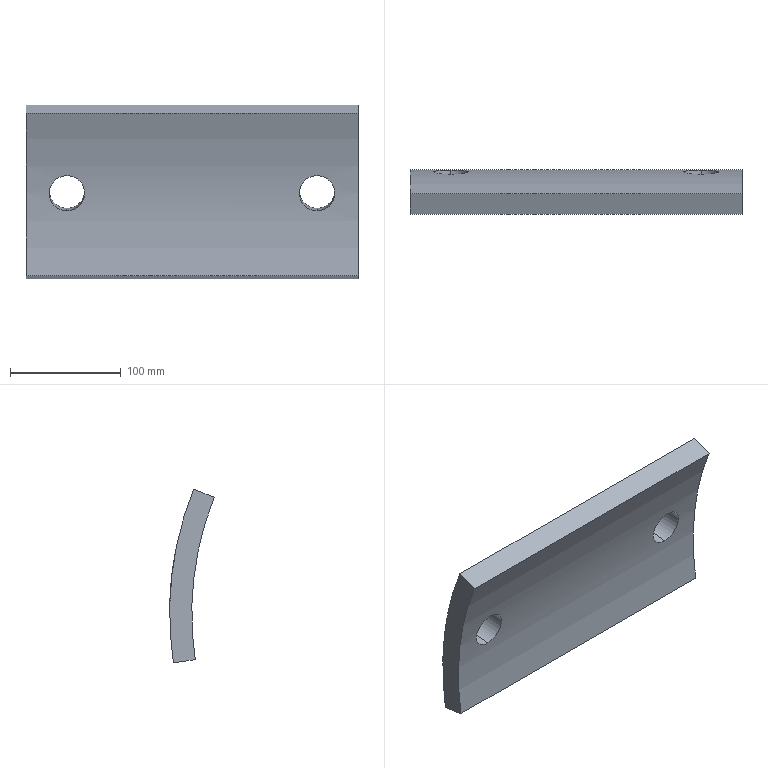Component | SolidWorks | Donja ploca spone-2 | 1 solid | 10 faces | box 300 x 40.3 x 157.04 mm | volume 895871 mm3 | cylinder 6 | plane 4 | commonest cylinder face diameters 32 x4 601 x1 561 x1
build123d program:
from build123d import *

# Parameters (mm, degrees)
BOSS_EXTRUDE1_DEPTH      = 150
BOSS_EXTRUDE1_DEPTH_BACK = 150
CUT_EXTRUDE3_DEPTH       = 171.734
CUT_EXTRUDE3_DEPTH_BACK  = 171.734
SKETCH2_R                = 16


with BuildPart() as part:
    # Sketch1 → Boss-Extrude1 (new, two sides: drawn at the far end of the back side and taken through both)
    with BuildSketch(Plane(origin=(0, 0, 0), x_dir=(0, 0, -1), z_dir=(1, 0, 0)).offset(-BOSS_EXTRUDE1_DEPTH_BACK)):
        with BuildLine():
            Line((-73.797, -9.882), (-79.058, 9.414))
            ThreePointArc((-79.058, 9.414), (0, 20), (79.058, 9.414))
            Line((79.058, 9.414), (73.797, -9.882))
            ThreePointArc((73.797, -9.882), (0, 0), (-73.797, -9.882))
        make_face()
    extrude(amount=BOSS_EXTRUDE1_DEPTH + BOSS_EXTRUDE1_DEPTH_BACK)

    # Sketch2 → Cut-Extrude3 (cut, two sides: drawn at the far end of the back side and taken through both)
    with BuildSketch(Plane(origin=(0, 0, 0), x_dir=(1, 0, 0), z_dir=(0, 1, 0)).offset(-CUT_EXTRUDE3_DEPTH_BACK)):
        with Locations(Location((113, 0, 0), (0, 0, 90))):
            Circle(SKETCH2_R)
        with Locations(Location((-113, 0, 0), (0, 0, 90))):
            Circle(SKETCH2_R)
    extrude(amount=CUT_EXTRUDE3_DEPTH + CUT_EXTRUDE3_DEPTH_BACK, mode=Mode.SUBTRACT)


solid = part.part

# Placed as in the assembly
solid = solid.moved(Location((-80, 278.597, 32.617), (6.678, 0, 0)))
STEP:
#1=CARTESIAN_POINT('',(-7.598,11.661,1.999));
#2=VERTEX_POINT('',#1);
#3=CARTESIAN_POINT('',(-7.598,11.807,0.7481));
#4=VERTEX_POINT('',#3);
#5=CARTESIAN_POINT('',(-7.598,11.661,1.999));
#6=CARTESIAN_POINT('',(-7.64,11.661,1.999));
#7=CARTESIAN_POINT('',(-7.68,11.661,1.995));
#8=CARTESIAN_POINT('',(-7.741,11.663,1.984));
#9=CARTESIAN_POINT('',(-7.762,11.664,1.979));
#10=CARTESIAN_POINT('',(-7.801,11.666,1.967));
#11=CARTESIAN_POINT('',(-7.84,11.668,1.953));
#12=CARTESIAN_POINT('',(-7.877,11.671,1.936));
#13=CARTESIAN_POINT('',(-7.913,11.674,1.917));
#14=CARTESIAN_POINT('',(-7.931,11.676,1.906));
#15=CARTESIAN_POINT('',(-7.983,11.682,1.872));
#16=CARTESIAN_POINT('',(-8.014,11.686,1.846));
#17=CARTESIAN_POINT('',(-8.058,11.693,1.803));
#18=CARTESIAN_POINT('',(-8.072,11.695,1.788));
#19=CARTESIAN_POINT('',(-8.098,11.7,1.756));
#20=CARTESIAN_POINT('',(-8.111,11.702,1.74));
#21=CARTESIAN_POINT('',(-8.145,11.71,1.689));
#22=CARTESIAN_POINT('',(-8.164,11.715,1.653));
#23=CARTESIAN_POINT('',(-8.188,11.723,1.597));
#24=CARTESIAN_POINT('',(-8.195,11.725,1.577));
#25=CARTESIAN_POINT('',(-8.207,11.73,1.538));
#26=CARTESIAN_POINT('',(-8.212,11.733,1.518));
#27=CARTESIAN_POINT('',(-8.224,11.741,1.458));
#28=CARTESIAN_POINT('',(-8.228,11.746,1.417));
#29=CARTESIAN_POINT('',(-8.228,11.753,1.356));
#30=CARTESIAN_POINT('',(-8.227,11.755,1.335));
#31=CARTESIAN_POINT('',(-8.223,11.76,1.294));
#32=CARTESIAN_POINT('',(-8.22,11.762,1.274));
#33=CARTESIAN_POINT('',(-8.212,11.766,1.234));
#34=CARTESIAN_POINT('',(-8.207,11.768,1.214));
#35=CARTESIAN_POINT('',(-8.195,11.772,1.175));
#36=CARTESIAN_POINT('',(-8.188,11.774,1.155));
#37=CARTESIAN_POINT('',(-8.165,11.78,1.098));
#38=CARTESIAN_POINT('',(-8.145,11.783,1.062));
#39=CARTESIAN_POINT('',(-8.111,11.787,1.011));
#40=CARTESIAN_POINT('',(-8.099,11.789,0.9945));
#41=CARTESIAN_POINT('',(-8.073,11.792,0.9624));
#42=CARTESIAN_POINT('',(-8.059,11.793,0.9472));
#43=CARTESIAN_POINT('',(-8.015,11.796,0.9036));
#44=CARTESIAN_POINT('',(-7.983,11.798,0.8776));
#45=CARTESIAN_POINT('',(-7.932,11.801,0.8431));
#46=CARTESIAN_POINT('',(-7.914,11.801,0.8324));
#47=CARTESIAN_POINT('',(-7.878,11.803,0.8129));
#48=CARTESIAN_POINT('',(-7.84,11.804,0.7954));
#49=CARTESIAN_POINT('',(-7.802,11.805,0.7815));
#50=CARTESIAN_POINT('',(-7.762,11.806,0.7695));
#51=CARTESIAN_POINT('',(-7.742,11.806,0.7644));
#52=CARTESIAN_POINT('',(-7.681,11.807,0.7522));
#53=CARTESIAN_POINT('',(-7.64,11.807,0.7481));
#54=CARTESIAN_POINT('',(-7.598,11.807,0.7481));
#55=B_SPLINE_CURVE_WITH_KNOTS('',3,(#5,#6,#7,#8,#9,#10,#11,#12,#13,#14,#15,#16,#17,#18,#19,#20,#21,#22,#23,#24,#25,#26,#27,#28,#29,#30,#31,#32,#33,#34,#35,#36,#37,#38,#39,#40,#41,#42,#43,#44,#45,#46,#47,#48,#49,#50,#51,#52,#53,#54),.UNSPECIFIED.,.F.,.F.,(4,2,2,1,2,2,2,2,2,2,2,2,2,2,2,2,2,2,2,2,2,2,1,2,2,4),(0.05003,0.05316,0.05472,0.05628,0.05785,0.05941,0.06254,0.0641,0.06566,0.06879,0.07035,0.07192,0.07504,0.07661,0.07817,0.07973,0.0813,0.08442,0.08598,0.08755,0.09067,0.09224,0.0938,0.09536,0.09693,0.1001),.UNSPECIFIED.);
#56=EDGE_CURVE('',#2,#4,#55,.T.);
#57=ORIENTED_EDGE('',*,*,#56,.F.);
#58=CARTESIAN_POINT('',(-7.598,10.877,1.908));
#59=VERTEX_POINT('',#58);
#60=CARTESIAN_POINT('',(-7.598,11.677,2.001));
#61=DIRECTION('',(0.,-0.9932,-0.1163));
#62=VECTOR('',#61,39.37);
#63=LINE('',#60,#62);
#64=EDGE_CURVE('',#2,#59,#63,.T.);
#65=ORIENTED_EDGE('',*,*,#64,.T.);
#66=CARTESIAN_POINT('',(-7.598,11.024,0.6564));
#67=VERTEX_POINT('',#66);
#68=CARTESIAN_POINT('',(-7.598,11.024,0.6564));
#69=CARTESIAN_POINT('',(-7.64,11.024,0.6564));
#70=CARTESIAN_POINT('',(-7.681,11.024,0.6605));
#71=CARTESIAN_POINT('',(-7.741,11.023,0.6725));
#72=CARTESIAN_POINT('',(-7.761,11.023,0.6775));
#73=CARTESIAN_POINT('',(-7.801,11.022,0.6895));
#74=CARTESIAN_POINT('',(-7.821,11.021,0.6965));
#75=CARTESIAN_POINT('',(-7.878,11.02,0.7202));
#76=CARTESIAN_POINT('',(-7.914,11.019,0.7396));
#77=CARTESIAN_POINT('',(-7.965,11.016,0.7738));
#78=CARTESIAN_POINT('',(-7.982,11.015,0.7862));
#79=CARTESIAN_POINT('',(-8.014,11.013,0.8125));
#80=CARTESIAN_POINT('',(-8.029,11.012,0.8263));
#81=CARTESIAN_POINT('',(-8.073,11.009,0.8698));
#82=CARTESIAN_POINT('',(-8.099,11.007,0.9014));
#83=CARTESIAN_POINT('',(-8.134,11.002,0.9529));
#84=CARTESIAN_POINT('',(-8.144,11.001,0.9707));
#85=CARTESIAN_POINT('',(-8.164,10.997,1.007));
#86=CARTESIAN_POINT('',(-8.181,10.994,1.044));
#87=CARTESIAN_POINT('',(-8.195,10.99,1.082));
#88=CARTESIAN_POINT('',(-8.207,10.986,1.122));
#89=CARTESIAN_POINT('',(-8.212,10.984,1.142));
#90=CARTESIAN_POINT('',(-8.224,10.978,1.202));
#91=CARTESIAN_POINT('',(-8.228,10.973,1.243));
#92=CARTESIAN_POINT('',(-8.228,10.966,1.304));
#93=CARTESIAN_POINT('',(-8.227,10.964,1.325));
#94=CARTESIAN_POINT('',(-8.223,10.959,1.366));
#95=CARTESIAN_POINT('',(-8.22,10.956,1.386));
#96=CARTESIAN_POINT('',(-8.208,10.948,1.446));
#97=CARTESIAN_POINT('',(-8.196,10.943,1.485));
#98=CARTESIAN_POINT('',(-8.173,10.935,1.542));
#99=CARTESIAN_POINT('',(-8.164,10.932,1.561));
#100=CARTESIAN_POINT('',(-8.144,10.927,1.597));
#101=CARTESIAN_POINT('',(-8.134,10.925,1.614));
#102=CARTESIAN_POINT('',(-8.099,10.917,1.665));
#103=CARTESIAN_POINT('',(-8.073,10.912,1.696));
#104=CARTESIAN_POINT('',(-8.015,10.903,1.754));
#105=CARTESIAN_POINT('',(-7.983,10.899,1.78));
#106=CARTESIAN_POINT('',(-7.932,10.893,1.814));
#107=CARTESIAN_POINT('',(-7.914,10.892,1.825));
#108=CARTESIAN_POINT('',(-7.877,10.888,1.844));
#109=CARTESIAN_POINT('',(-7.859,10.887,1.853));
#110=CARTESIAN_POINT('',(-7.801,10.883,1.876));
#111=CARTESIAN_POINT('',(-7.762,10.881,1.888));
#112=CARTESIAN_POINT('',(-7.701,10.879,1.9));
#113=CARTESIAN_POINT('',(-7.681,10.878,1.903));
#114=CARTESIAN_POINT('',(-7.64,10.877,1.907));
#115=CARTESIAN_POINT('',(-7.619,10.877,1.908));
#116=CARTESIAN_POINT('',(-7.598,10.877,1.908));
#117=B_SPLINE_CURVE_WITH_KNOTS('',3,(#68,#69,#70,#71,#72,#73,#74,#75,#76,#77,#78,#79,#80,#81,#82,#83,#84,#85,#86,#87,#88,#89,#90,#91,#92,#93,#94,#95,#96,#97,#98,#99,#100,#101,#102,#103,#104,#105,#106,#107,#108,#109,#110,#111,#112,#113,#114,#115,#116),.UNSPECIFIED.,.F.,.F.,(4,2,2,2,2,2,2,2,2,1,2,2,2,2,2,2,2,2,2,2,2,2,2,2,4),(0.,0.003127,0.004691,0.006254,0.009381,0.01094,0.01251,0.01564,0.0172,0.01876,0.02033,0.02189,0.02502,0.02658,0.02814,0.03127,0.03283,0.0344,0.03753,0.04065,0.04222,0.04378,0.04691,0.04847,0.05003),.UNSPECIFIED.);
#118=EDGE_CURVE('',#67,#59,#117,.T.);
#119=ORIENTED_EDGE('',*,*,#118,.F.);
#120=CARTESIAN_POINT('',(-7.598,11.824,0.7501));
#121=DIRECTION('',(0.,-0.9932,-0.1163));
#122=VECTOR('',#121,39.37);
#123=LINE('',#120,#122);
#124=EDGE_CURVE('',#4,#67,#123,.T.);
#125=ORIENTED_EDGE('',*,*,#124,.F.);
#126=EDGE_LOOP('',(#57,#65,#119,#125));
#127=FACE_OUTER_BOUND('',#126,.T.);
#128=CARTESIAN_POINT('',(-7.598,11.75,1.376));
#129=DIRECTION('',(0.,-0.9932,-0.1163));
#130=DIRECTION('',(0.,0.1163,-0.9932));
#131=AXIS2_PLACEMENT_3D('',#128,#129,#130);
#132=CYLINDRICAL_SURFACE('',#131,0.6299);
#133=ADVANCED_FACE('',(#127),#132,.F.);
#134=CARTESIAN_POINT('',(1.299,11.661,1.999));
#135=VERTEX_POINT('',#134);
#136=CARTESIAN_POINT('',(1.299,11.807,0.7481));
#137=VERTEX_POINT('',#136);
#138=CARTESIAN_POINT('',(1.299,11.661,1.999));
#139=CARTESIAN_POINT('',(1.258,11.661,1.999));
#140=CARTESIAN_POINT('',(1.217,11.661,1.995));
#141=CARTESIAN_POINT('',(1.156,11.663,1.984));
#142=CARTESIAN_POINT('',(1.136,11.664,1.979));
#143=CARTESIAN_POINT('',(1.097,11.666,1.967));
#144=CARTESIAN_POINT('',(1.058,11.668,1.953));
#145=CARTESIAN_POINT('',(1.021,11.671,1.936));
#146=CARTESIAN_POINT('',(0.9845,11.674,1.917));
#147=CARTESIAN_POINT('',(0.9666,11.676,1.906));
#148=CARTESIAN_POINT('',(0.9149,11.682,1.872));
#149=CARTESIAN_POINT('',(0.8832,11.686,1.846));
#150=CARTESIAN_POINT('',(0.8396,11.693,1.803));
#151=CARTESIAN_POINT('',(0.8257,11.695,1.788));
#152=CARTESIAN_POINT('',(0.7994,11.7,1.756));
#153=CARTESIAN_POINT('',(0.787,11.702,1.74));
#154=CARTESIAN_POINT('',(0.7527,11.71,1.689));
#155=CARTESIAN_POINT('',(0.7333,11.715,1.653));
#156=CARTESIAN_POINT('',(0.7096,11.723,1.597));
#157=CARTESIAN_POINT('',(0.7025,11.725,1.577));
#158=CARTESIAN_POINT('',(0.6905,11.73,1.538));
#159=CARTESIAN_POINT('',(0.6855,11.733,1.518));
#160=CARTESIAN_POINT('',(0.6734,11.741,1.458));
#161=CARTESIAN_POINT('',(0.6693,11.746,1.417));
#162=CARTESIAN_POINT('',(0.6693,11.753,1.356));
#163=CARTESIAN_POINT('',(0.6703,11.755,1.335));
#164=CARTESIAN_POINT('',(0.6743,11.76,1.294));
#165=CARTESIAN_POINT('',(0.6773,11.762,1.274));
#166=CARTESIAN_POINT('',(0.6853,11.766,1.234));
#167=CARTESIAN_POINT('',(0.6902,11.768,1.214));
#168=CARTESIAN_POINT('',(0.7022,11.772,1.175));
#169=CARTESIAN_POINT('',(0.7092,11.774,1.155));
#170=CARTESIAN_POINT('',(0.7329,11.78,1.098));
#171=CARTESIAN_POINT('',(0.7522,11.783,1.062));
#172=CARTESIAN_POINT('',(0.7864,11.787,1.011));
#173=CARTESIAN_POINT('',(0.7987,11.789,0.9945));
#174=CARTESIAN_POINT('',(0.8251,11.792,0.9624));
#175=CARTESIAN_POINT('',(0.839,11.793,0.9472));
#176=CARTESIAN_POINT('',(0.8825,11.796,0.9036));
#177=CARTESIAN_POINT('',(0.9142,11.798,0.8776));
#178=CARTESIAN_POINT('',(0.9657,11.801,0.8431));
#179=CARTESIAN_POINT('',(0.9836,11.801,0.8324));
#180=CARTESIAN_POINT('',(1.02,11.803,0.8129));
#181=CARTESIAN_POINT('',(1.057,11.804,0.7954));
#182=CARTESIAN_POINT('',(1.096,11.805,0.7815));
#183=CARTESIAN_POINT('',(1.135,11.806,0.7695));
#184=CARTESIAN_POINT('',(1.155,11.806,0.7644));
#185=CARTESIAN_POINT('',(1.216,11.807,0.7522));
#186=CARTESIAN_POINT('',(1.258,11.807,0.7481));
#187=CARTESIAN_POINT('',(1.299,11.807,0.7481));
#188=B_SPLINE_CURVE_WITH_KNOTS('',3,(#138,#139,#140,#141,#142,#143,#144,#145,#146,#147,#148,#149,#150,#151,#152,#153,#154,#155,#156,#157,#158,#159,#160,#161,#162,#163,#164,#165,#166,#167,#168,#169,#170,#171,#172,#173,#174,#175,#176,#177,#178,#179,#180,#181,#182,#183,#184,#185,#186,#187),.UNSPECIFIED.,.F.,.F.,(4,2,2,1,2,2,2,2,2,2,2,2,2,2,2,2,2,2,2,2,2,2,1,2,2,4),(0.05003,0.05316,0.05472,0.05628,0.05785,0.05941,0.06254,0.0641,0.06566,0.06879,0.07035,0.07192,0.07504,0.07661,0.07817,0.07973,0.0813,0.08442,0.08598,0.08755,0.09067,0.09224,0.0938,0.09536,0.09693,0.1001),.UNSPECIFIED.);
#189=EDGE_CURVE('',#135,#137,#188,.T.);
#190=ORIENTED_EDGE('',*,*,#189,.F.);
#191=CARTESIAN_POINT('',(1.299,10.877,1.908));
#192=VERTEX_POINT('',#191);
#193=CARTESIAN_POINT('',(1.299,11.677,2.001));
#194=DIRECTION('',(0.,-0.9932,-0.1163));
#195=VECTOR('',#194,39.37);
#196=LINE('',#193,#195);
#197=EDGE_CURVE('',#135,#192,#196,.T.);
#198=ORIENTED_EDGE('',*,*,#197,.T.);
#199=CARTESIAN_POINT('',(1.299,11.024,0.6564));
#200=VERTEX_POINT('',#199);
#201=CARTESIAN_POINT('',(1.299,11.024,0.6564));
#202=CARTESIAN_POINT('',(1.258,11.024,0.6564));
#203=CARTESIAN_POINT('',(1.217,11.024,0.6605));
#204=CARTESIAN_POINT('',(1.156,11.023,0.6725));
#205=CARTESIAN_POINT('',(1.136,11.023,0.6775));
#206=CARTESIAN_POINT('',(1.097,11.022,0.6895));
#207=CARTESIAN_POINT('',(1.077,11.021,0.6965));
#208=CARTESIAN_POINT('',(1.02,11.02,0.7202));
#209=CARTESIAN_POINT('',(0.9836,11.019,0.7396));
#210=CARTESIAN_POINT('',(0.9323,11.016,0.7738));
#211=CARTESIAN_POINT('',(0.9156,11.015,0.7862));
#212=CARTESIAN_POINT('',(0.8835,11.013,0.8125));
#213=CARTESIAN_POINT('',(0.8682,11.012,0.8263));
#214=CARTESIAN_POINT('',(0.8247,11.009,0.8698));
#215=CARTESIAN_POINT('',(0.7986,11.007,0.9014));
#216=CARTESIAN_POINT('',(0.7641,11.002,0.9529));
#217=CARTESIAN_POINT('',(0.7533,11.001,0.9707));
#218=CARTESIAN_POINT('',(0.7339,10.997,1.007));
#219=CARTESIAN_POINT('',(0.7163,10.994,1.044));
#220=CARTESIAN_POINT('',(0.7025,10.99,1.082));
#221=CARTESIAN_POINT('',(0.6905,10.986,1.122));
#222=CARTESIAN_POINT('',(0.6854,10.984,1.142));
#223=CARTESIAN_POINT('',(0.6733,10.978,1.202));
#224=CARTESIAN_POINT('',(0.6693,10.973,1.243));
#225=CARTESIAN_POINT('',(0.6693,10.966,1.304));
#226=CARTESIAN_POINT('',(0.6703,10.964,1.325));
#227=CARTESIAN_POINT('',(0.6743,10.959,1.366));
#228=CARTESIAN_POINT('',(0.6774,10.956,1.386));
#229=CARTESIAN_POINT('',(0.6895,10.948,1.446));
#230=CARTESIAN_POINT('',(0.7014,10.943,1.485));
#231=CARTESIAN_POINT('',(0.725,10.935,1.542));
#232=CARTESIAN_POINT('',(0.734,10.932,1.561));
#233=CARTESIAN_POINT('',(0.7535,10.927,1.597));
#234=CARTESIAN_POINT('',(0.7641,10.925,1.614));
#235=CARTESIAN_POINT('',(0.7983,10.917,1.665));
#236=CARTESIAN_POINT('',(0.8243,10.912,1.696));
#237=CARTESIAN_POINT('',(0.8831,10.903,1.754));
#238=CARTESIAN_POINT('',(0.915,10.899,1.78));
#239=CARTESIAN_POINT('',(0.9661,10.893,1.814));
#240=CARTESIAN_POINT('',(0.9838,10.892,1.825));
#241=CARTESIAN_POINT('',(1.02,10.888,1.844));
#242=CARTESIAN_POINT('',(1.039,10.887,1.853));
#243=CARTESIAN_POINT('',(1.096,10.883,1.876));
#244=CARTESIAN_POINT('',(1.136,10.881,1.888));
#245=CARTESIAN_POINT('',(1.196,10.879,1.9));
#246=CARTESIAN_POINT('',(1.217,10.878,1.903));
#247=CARTESIAN_POINT('',(1.258,10.877,1.907));
#248=CARTESIAN_POINT('',(1.279,10.877,1.908));
#249=CARTESIAN_POINT('',(1.299,10.877,1.908));
#250=B_SPLINE_CURVE_WITH_KNOTS('',3,(#201,#202,#203,#204,#205,#206,#207,#208,#209,#210,#211,#212,#213,#214,#215,#216,#217,#218,#219,#220,#221,#222,#223,#224,#225,#226,#227,#228,#229,#230,#231,#232,#233,#234,#235,#236,#237,#238,#239,#240,#241,#242,#243,#244,#245,#246,#247,#248,#249),.UNSPECIFIED.,.F.,.F.,(4,2,2,2,2,2,2,2,2,1,2,2,2,2,2,2,2,2,2,2,2,2,2,2,4),(0.,0.003127,0.004691,0.006254,0.009381,0.01094,0.01251,0.01564,0.0172,0.01876,0.02033,0.02189,0.02502,0.02658,0.02814,0.03127,0.03283,0.0344,0.03753,0.04065,0.04222,0.04378,0.04691,0.04847,0.05003),.UNSPECIFIED.);
#251=EDGE_CURVE('',#200,#192,#250,.T.);
#252=ORIENTED_EDGE('',*,*,#251,.F.);
#253=CARTESIAN_POINT('',(1.299,11.824,0.7501));
#254=DIRECTION('',(0.,-0.9932,-0.1163));
#255=VECTOR('',#254,39.37);
#256=LINE('',#253,#255);
#257=EDGE_CURVE('',#137,#200,#256,.T.);
#258=ORIENTED_EDGE('',*,*,#257,.F.);
#259=EDGE_LOOP('',(#190,#198,#252,#258));
#260=FACE_OUTER_BOUND('',#259,.T.);
#261=CARTESIAN_POINT('',(1.299,11.75,1.376));
#262=DIRECTION('',(0.,-0.9932,-0.1163));
#263=DIRECTION('',(0.,0.1163,-0.9932));
#264=AXIS2_PLACEMENT_3D('',#261,#262,#263);
#265=CYLINDRICAL_SURFACE('',#264,0.6299);
#266=ADVANCED_FACE('',(#260),#265,.F.);
#267=CARTESIAN_POINT('',(-9.055,10.975,4.419));
#268=VERTEX_POINT('',#267);
#269=CARTESIAN_POINT('',(2.756,10.975,4.419));
#270=VERTEX_POINT('',#269);
#271=CARTESIAN_POINT('',(-9.055,10.975,4.419));
#272=DIRECTION('',(1.,0.,0.));
#273=VECTOR('',#272,39.37);
#274=LINE('',#271,#273);
#275=EDGE_CURVE('',#268,#270,#274,.T.);
#276=ORIENTED_EDGE('',*,*,#275,.T.);
#277=CARTESIAN_POINT('',(2.756,11.698,-1.764));
#278=VERTEX_POINT('',#277);
#279=CARTESIAN_POINT('',(2.756,0.,0.));
#280=DIRECTION('',(1.,0.,0.));
#281=DIRECTION('',(0.,0.1163,-0.9932));
#282=AXIS2_PLACEMENT_3D('',#279,#280,#281);
#283=CIRCLE('',#282,11.831);
#284=EDGE_CURVE('',#278,#270,#283,.T.);
#285=ORIENTED_EDGE('',*,*,#284,.F.);
#286=CARTESIAN_POINT('',(-9.055,11.698,-1.764));
#287=VERTEX_POINT('',#286);
#288=CARTESIAN_POINT('',(-9.055,11.698,-1.764));
#289=DIRECTION('',(1.,0.,0.));
#290=VECTOR('',#289,39.37);
#291=LINE('',#288,#290);
#292=EDGE_CURVE('',#287,#278,#291,.T.);
#293=ORIENTED_EDGE('',*,*,#292,.F.);
#294=CARTESIAN_POINT('',(-9.055,0.,0.));
#295=DIRECTION('',(1.,0.,0.));
#296=DIRECTION('',(0.,0.1163,-0.9932));
#297=AXIS2_PLACEMENT_3D('',#294,#295,#296);
#298=CIRCLE('',#297,11.831);
#299=EDGE_CURVE('',#287,#268,#298,.T.);
#300=ORIENTED_EDGE('',*,*,#299,.T.);
#301=EDGE_LOOP('',(#276,#285,#293,#300));
#302=FACE_OUTER_BOUND('',#301,.T.);
#303=CARTESIAN_POINT('',(1.299,11.807,0.7481));
#304=CARTESIAN_POINT('',(1.341,11.807,0.7481));
#305=CARTESIAN_POINT('',(1.382,11.807,0.7522));
#306=CARTESIAN_POINT('',(1.442,11.806,0.7642));
#307=CARTESIAN_POINT('',(1.462,11.806,0.7692));
#308=CARTESIAN_POINT('',(1.502,11.805,0.7812));
#309=CARTESIAN_POINT('',(1.521,11.804,0.7882));
#310=CARTESIAN_POINT('',(1.579,11.803,0.8119));
#311=CARTESIAN_POINT('',(1.615,11.801,0.8312));
#312=CARTESIAN_POINT('',(1.666,11.799,0.8655));
#313=CARTESIAN_POINT('',(1.683,11.798,0.8778));
#314=CARTESIAN_POINT('',(1.715,11.796,0.9041));
#315=CARTESIAN_POINT('',(1.73,11.795,0.9179));
#316=CARTESIAN_POINT('',(1.774,11.792,0.9614));
#317=CARTESIAN_POINT('',(1.8,11.789,0.993));
#318=CARTESIAN_POINT('',(1.834,11.785,1.045));
#319=CARTESIAN_POINT('',(1.845,11.783,1.062));
#320=CARTESIAN_POINT('',(1.865,11.78,1.099));
#321=CARTESIAN_POINT('',(1.882,11.776,1.136));
#322=CARTESIAN_POINT('',(1.896,11.772,1.174));
#323=CARTESIAN_POINT('',(1.908,11.768,1.213));
#324=CARTESIAN_POINT('',(1.913,11.766,1.233));
#325=CARTESIAN_POINT('',(1.925,11.76,1.294));
#326=CARTESIAN_POINT('',(1.929,11.755,1.335));
#327=CARTESIAN_POINT('',(1.929,11.748,1.396));
#328=CARTESIAN_POINT('',(1.928,11.746,1.416));
#329=CARTESIAN_POINT('',(1.924,11.741,1.457));
#330=CARTESIAN_POINT('',(1.921,11.738,1.478));
#331=CARTESIAN_POINT('',(1.909,11.73,1.538));
#332=CARTESIAN_POINT('',(1.897,11.725,1.577));
#333=CARTESIAN_POINT('',(1.873,11.717,1.634));
#334=CARTESIAN_POINT('',(1.864,11.715,1.652));
#335=CARTESIAN_POINT('',(1.845,11.71,1.688));
#336=CARTESIAN_POINT('',(1.834,11.707,1.706));
#337=CARTESIAN_POINT('',(1.8,11.7,1.756));
#338=CARTESIAN_POINT('',(1.774,11.695,1.788));
#339=CARTESIAN_POINT('',(1.715,11.686,1.846));
#340=CARTESIAN_POINT('',(1.683,11.682,1.872));
#341=CARTESIAN_POINT('',(1.632,11.676,1.906));
#342=CARTESIAN_POINT('',(1.615,11.675,1.916));
#343=CARTESIAN_POINT('',(1.578,11.671,1.935));
#344=CARTESIAN_POINT('',(1.559,11.67,1.944));
#345=CARTESIAN_POINT('',(1.502,11.666,1.968));
#346=CARTESIAN_POINT('',(1.463,11.664,1.979));
#347=CARTESIAN_POINT('',(1.402,11.662,1.991));
#348=CARTESIAN_POINT('',(1.382,11.661,1.994));
#349=CARTESIAN_POINT('',(1.34,11.661,1.998));
#350=CARTESIAN_POINT('',(1.32,11.661,1.999));
#351=CARTESIAN_POINT('',(1.299,11.661,1.999));
#352=B_SPLINE_CURVE_WITH_KNOTS('',3,(#303,#304,#305,#306,#307,#308,#309,#310,#311,#312,#313,#314,#315,#316,#317,#318,#319,#320,#321,#322,#323,#324,#325,#326,#327,#328,#329,#330,#331,#332,#333,#334,#335,#336,#337,#338,#339,#340,#341,#342,#343,#344,#345,#346,#347,#348,#349,#350,#351),.UNSPECIFIED.,.F.,.F.,(4,2,2,2,2,2,2,2,2,1,2,2,2,2,2,2,2,2,2,2,2,2,2,2,4),(0.,0.003127,0.004691,0.006254,0.009381,0.01094,0.01251,0.01564,0.0172,0.01876,0.02033,0.02189,0.02502,0.02658,0.02814,0.03127,0.03283,0.0344,0.03752,0.04065,0.04221,0.04378,0.04691,0.04847,0.05003),.UNSPECIFIED.);
#353=EDGE_CURVE('',#137,#135,#352,.T.);
#354=ORIENTED_EDGE('',*,*,#353,.T.);
#355=ORIENTED_EDGE('',*,*,#189,.T.);
#356=EDGE_LOOP('',(#354,#355));
#357=FACE_BOUND('',#356,.T.);
#358=CARTESIAN_POINT('',(-7.598,11.807,0.7481));
#359=CARTESIAN_POINT('',(-7.557,11.807,0.7481));
#360=CARTESIAN_POINT('',(-7.516,11.807,0.7522));
#361=CARTESIAN_POINT('',(-7.455,11.806,0.7642));
#362=CARTESIAN_POINT('',(-7.436,11.806,0.7692));
#363=CARTESIAN_POINT('',(-7.396,11.805,0.7812));
#364=CARTESIAN_POINT('',(-7.376,11.804,0.7882));
#365=CARTESIAN_POINT('',(-7.319,11.803,0.8119));
#366=CARTESIAN_POINT('',(-7.283,11.801,0.8312));
#367=CARTESIAN_POINT('',(-7.232,11.799,0.8655));
#368=CARTESIAN_POINT('',(-7.215,11.798,0.8778));
#369=CARTESIAN_POINT('',(-7.183,11.796,0.9041));
#370=CARTESIAN_POINT('',(-7.167,11.795,0.9179));
#371=CARTESIAN_POINT('',(-7.124,11.792,0.9614));
#372=CARTESIAN_POINT('',(-7.098,11.789,0.993));
#373=CARTESIAN_POINT('',(-7.063,11.785,1.045));
#374=CARTESIAN_POINT('',(-7.053,11.783,1.062));
#375=CARTESIAN_POINT('',(-7.033,11.78,1.099));
#376=CARTESIAN_POINT('',(-7.016,11.776,1.136));
#377=CARTESIAN_POINT('',(-7.002,11.772,1.174));
#378=CARTESIAN_POINT('',(-6.99,11.768,1.213));
#379=CARTESIAN_POINT('',(-6.985,11.766,1.233));
#380=CARTESIAN_POINT('',(-6.973,11.76,1.294));
#381=CARTESIAN_POINT('',(-6.969,11.755,1.335));
#382=CARTESIAN_POINT('',(-6.968,11.748,1.396));
#383=CARTESIAN_POINT('',(-6.969,11.746,1.416));
#384=CARTESIAN_POINT('',(-6.974,11.741,1.457));
#385=CARTESIAN_POINT('',(-6.977,11.738,1.478));
#386=CARTESIAN_POINT('',(-6.989,11.73,1.538));
#387=CARTESIAN_POINT('',(-7.001,11.725,1.577));
#388=CARTESIAN_POINT('',(-7.024,11.717,1.634));
#389=CARTESIAN_POINT('',(-7.033,11.715,1.652));
#390=CARTESIAN_POINT('',(-7.053,11.71,1.688));
#391=CARTESIAN_POINT('',(-7.063,11.707,1.706));
#392=CARTESIAN_POINT('',(-7.097,11.7,1.756));
#393=CARTESIAN_POINT('',(-7.124,11.695,1.788));
#394=CARTESIAN_POINT('',(-7.182,11.686,1.846));
#395=CARTESIAN_POINT('',(-7.214,11.682,1.872));
#396=CARTESIAN_POINT('',(-7.265,11.676,1.906));
#397=CARTESIAN_POINT('',(-7.283,11.675,1.916));
#398=CARTESIAN_POINT('',(-7.319,11.671,1.935));
#399=CARTESIAN_POINT('',(-7.338,11.67,1.944));
#400=CARTESIAN_POINT('',(-7.396,11.666,1.968));
#401=CARTESIAN_POINT('',(-7.435,11.664,1.979));
#402=CARTESIAN_POINT('',(-7.495,11.662,1.991));
#403=CARTESIAN_POINT('',(-7.516,11.661,1.994));
#404=CARTESIAN_POINT('',(-7.557,11.661,1.998));
#405=CARTESIAN_POINT('',(-7.578,11.661,1.999));
#406=CARTESIAN_POINT('',(-7.598,11.661,1.999));
#407=B_SPLINE_CURVE_WITH_KNOTS('',3,(#358,#359,#360,#361,#362,#363,#364,#365,#366,#367,#368,#369,#370,#371,#372,#373,#374,#375,#376,#377,#378,#379,#380,#381,#382,#383,#384,#385,#386,#387,#388,#389,#390,#391,#392,#393,#394,#395,#396,#397,#398,#399,#400,#401,#402,#403,#404,#405,#406),.UNSPECIFIED.,.F.,.F.,(4,2,2,2,2,2,2,2,2,1,2,2,2,2,2,2,2,2,2,2,2,2,2,2,4),(0.,0.003127,0.004691,0.006254,0.009381,0.01094,0.01251,0.01564,0.0172,0.01876,0.02033,0.02189,0.02502,0.02658,0.02814,0.03127,0.03283,0.0344,0.03752,0.04065,0.04221,0.04378,0.04691,0.04847,0.05003),.UNSPECIFIED.);
#408=EDGE_CURVE('',#4,#2,#407,.T.);
#409=ORIENTED_EDGE('',*,*,#408,.T.);
#410=ORIENTED_EDGE('',*,*,#56,.T.);
#411=EDGE_LOOP('',(#409,#410));
#412=FACE_BOUND('',#411,.T.);
#413=CARTESIAN_POINT('',(-9.055,0.,0.));
#414=DIRECTION('',(1.,0.,0.));
#415=DIRECTION('',(0.,0.1163,-0.9932));
#416=AXIS2_PLACEMENT_3D('',#413,#414,#415);
#417=CYLINDRICAL_SURFACE('',#416,11.831);
#418=ADVANCED_FACE('',(#302,#357,#412),#417,.T.);
#419=ORIENTED_EDGE('',*,*,#251,.T.);
#420=CARTESIAN_POINT('',(1.299,10.877,1.908));
#421=CARTESIAN_POINT('',(1.34,10.877,1.908));
#422=CARTESIAN_POINT('',(1.381,10.878,1.904));
#423=CARTESIAN_POINT('',(1.442,10.88,1.892));
#424=CARTESIAN_POINT('',(1.462,10.881,1.887));
#425=CARTESIAN_POINT('',(1.502,10.883,1.875));
#426=CARTESIAN_POINT('',(1.54,10.885,1.861));
#427=CARTESIAN_POINT('',(1.578,10.888,1.844));
#428=CARTESIAN_POINT('',(1.614,10.891,1.825));
#429=CARTESIAN_POINT('',(1.632,10.893,1.814));
#430=CARTESIAN_POINT('',(1.684,10.899,1.78));
#431=CARTESIAN_POINT('',(1.715,10.903,1.754));
#432=CARTESIAN_POINT('',(1.759,10.91,1.711));
#433=CARTESIAN_POINT('',(1.773,10.912,1.696));
#434=CARTESIAN_POINT('',(1.799,10.917,1.665));
#435=CARTESIAN_POINT('',(1.811,10.92,1.648));
#436=CARTESIAN_POINT('',(1.846,10.927,1.597));
#437=CARTESIAN_POINT('',(1.865,10.932,1.562));
#438=CARTESIAN_POINT('',(1.889,10.94,1.505));
#439=CARTESIAN_POINT('',(1.896,10.943,1.485));
#440=CARTESIAN_POINT('',(1.908,10.948,1.446));
#441=CARTESIAN_POINT('',(1.913,10.951,1.426));
#442=CARTESIAN_POINT('',(1.925,10.959,1.367));
#443=CARTESIAN_POINT('',(1.929,10.963,1.326));
#444=CARTESIAN_POINT('',(1.929,10.971,1.264));
#445=CARTESIAN_POINT('',(1.928,10.973,1.243));
#446=CARTESIAN_POINT('',(1.924,10.978,1.203));
#447=CARTESIAN_POINT('',(1.921,10.98,1.183));
#448=CARTESIAN_POINT('',(1.913,10.984,1.143));
#449=CARTESIAN_POINT('',(1.908,10.986,1.123));
#450=CARTESIAN_POINT('',(1.896,10.99,1.083));
#451=CARTESIAN_POINT('',(1.889,10.992,1.064));
#452=CARTESIAN_POINT('',(1.866,10.997,1.007));
#453=CARTESIAN_POINT('',(1.846,11.001,0.9706));
#454=CARTESIAN_POINT('',(1.812,11.005,0.9195));
#455=CARTESIAN_POINT('',(1.8,11.006,0.9029));
#456=CARTESIAN_POINT('',(1.773,11.009,0.8708));
#457=CARTESIAN_POINT('',(1.759,11.01,0.8555));
#458=CARTESIAN_POINT('',(1.716,11.013,0.812));
#459=CARTESIAN_POINT('',(1.684,11.015,0.786));
#460=CARTESIAN_POINT('',(1.633,11.018,0.7515));
#461=CARTESIAN_POINT('',(1.615,11.018,0.7407));
#462=CARTESIAN_POINT('',(1.578,11.02,0.7213));
#463=CARTESIAN_POINT('',(1.541,11.021,0.7037));
#464=CARTESIAN_POINT('',(1.503,11.022,0.6898));
#465=CARTESIAN_POINT('',(1.463,11.022,0.6778));
#466=CARTESIAN_POINT('',(1.443,11.023,0.6727));
#467=CARTESIAN_POINT('',(1.382,11.024,0.6605));
#468=CARTESIAN_POINT('',(1.341,11.024,0.6564));
#469=CARTESIAN_POINT('',(1.299,11.024,0.6564));
#470=B_SPLINE_CURVE_WITH_KNOTS('',3,(#420,#421,#422,#423,#424,#425,#426,#427,#428,#429,#430,#431,#432,#433,#434,#435,#436,#437,#438,#439,#440,#441,#442,#443,#444,#445,#446,#447,#448,#449,#450,#451,#452,#453,#454,#455,#456,#457,#458,#459,#460,#461,#462,#463,#464,#465,#466,#467,#468,#469),.UNSPECIFIED.,.F.,.F.,(4,2,2,1,2,2,2,2,2,2,2,2,2,2,2,2,2,2,2,2,2,2,1,2,2,4),(0.05003,0.05316,0.05472,0.05629,0.05785,0.05941,0.06254,0.0641,0.06567,0.06879,0.07035,0.07192,0.07504,0.07661,0.07817,0.07973,0.0813,0.08442,0.08599,0.08755,0.09068,0.09224,0.0938,0.09537,0.09693,0.1001),.UNSPECIFIED.);
#471=EDGE_CURVE('',#192,#200,#470,.T.);
#472=ORIENTED_EDGE('',*,*,#471,.T.);
#473=EDGE_LOOP('',(#419,#472));
#474=FACE_BOUND('',#473,.T.);
#475=CARTESIAN_POINT('',(-9.055,10.92,-1.647));
#476=VERTEX_POINT('',#475);
#477=CARTESIAN_POINT('',(2.756,10.92,-1.647));
#478=VERTEX_POINT('',#477);
#479=CARTESIAN_POINT('',(-9.055,10.92,-1.647));
#480=DIRECTION('',(1.,0.,0.));
#481=VECTOR('',#480,39.37);
#482=LINE('',#479,#481);
#483=EDGE_CURVE('',#476,#478,#482,.T.);
#484=ORIENTED_EDGE('',*,*,#483,.T.);
#485=CARTESIAN_POINT('',(2.756,10.244,4.125));
#486=VERTEX_POINT('',#485);
#487=CARTESIAN_POINT('',(2.756,0.,0.));
#488=DIRECTION('',(-1.,-0.,-0.));
#489=DIRECTION('',(0.,0.1163,-0.9932));
#490=AXIS2_PLACEMENT_3D('',#487,#488,#489);
#491=CIRCLE('',#490,11.043);
#492=EDGE_CURVE('',#486,#478,#491,.T.);
#493=ORIENTED_EDGE('',*,*,#492,.F.);
#494=CARTESIAN_POINT('',(-9.055,10.244,4.125));
#495=VERTEX_POINT('',#494);
#496=CARTESIAN_POINT('',(-9.055,10.244,4.125));
#497=DIRECTION('',(1.,0.,0.));
#498=VECTOR('',#497,39.37);
#499=LINE('',#496,#498);
#500=EDGE_CURVE('',#495,#486,#499,.T.);
#501=ORIENTED_EDGE('',*,*,#500,.F.);
#502=CARTESIAN_POINT('',(-9.055,0.,0.));
#503=DIRECTION('',(-1.,-0.,-0.));
#504=DIRECTION('',(0.,0.1163,-0.9932));
#505=AXIS2_PLACEMENT_3D('',#502,#503,#504);
#506=CIRCLE('',#505,11.043);
#507=EDGE_CURVE('',#495,#476,#506,.T.);
#508=ORIENTED_EDGE('',*,*,#507,.T.);
#509=EDGE_LOOP('',(#484,#493,#501,#508));
#510=FACE_OUTER_BOUND('',#509,.T.);
#511=ORIENTED_EDGE('',*,*,#118,.T.);
#512=CARTESIAN_POINT('',(-7.598,10.877,1.908));
#513=CARTESIAN_POINT('',(-7.557,10.877,1.908));
#514=CARTESIAN_POINT('',(-7.516,10.878,1.904));
#515=CARTESIAN_POINT('',(-7.456,10.88,1.892));
#516=CARTESIAN_POINT('',(-7.435,10.881,1.887));
#517=CARTESIAN_POINT('',(-7.396,10.883,1.875));
#518=CARTESIAN_POINT('',(-7.357,10.885,1.861));
#519=CARTESIAN_POINT('',(-7.32,10.888,1.844));
#520=CARTESIAN_POINT('',(-7.284,10.891,1.825));
#521=CARTESIAN_POINT('',(-7.266,10.893,1.814));
#522=CARTESIAN_POINT('',(-7.214,10.899,1.78));
#523=CARTESIAN_POINT('',(-7.182,10.903,1.754));
#524=CARTESIAN_POINT('',(-7.139,10.91,1.711));
#525=CARTESIAN_POINT('',(-7.125,10.912,1.696));
#526=CARTESIAN_POINT('',(-7.099,10.917,1.665));
#527=CARTESIAN_POINT('',(-7.086,10.92,1.648));
#528=CARTESIAN_POINT('',(-7.052,10.927,1.597));
#529=CARTESIAN_POINT('',(-7.033,10.932,1.562));
#530=CARTESIAN_POINT('',(-7.009,10.94,1.505));
#531=CARTESIAN_POINT('',(-7.002,10.943,1.485));
#532=CARTESIAN_POINT('',(-6.99,10.948,1.446));
#533=CARTESIAN_POINT('',(-6.985,10.951,1.426));
#534=CARTESIAN_POINT('',(-6.973,10.959,1.367));
#535=CARTESIAN_POINT('',(-6.969,10.963,1.326));
#536=CARTESIAN_POINT('',(-6.968,10.971,1.264));
#537=CARTESIAN_POINT('',(-6.97,10.973,1.243));
#538=CARTESIAN_POINT('',(-6.974,10.978,1.203));
#539=CARTESIAN_POINT('',(-6.977,10.98,1.183));
#540=CARTESIAN_POINT('',(-6.984,10.984,1.143));
#541=CARTESIAN_POINT('',(-6.989,10.986,1.123));
#542=CARTESIAN_POINT('',(-7.001,10.99,1.083));
#543=CARTESIAN_POINT('',(-7.008,10.992,1.064));
#544=CARTESIAN_POINT('',(-7.032,10.997,1.007));
#545=CARTESIAN_POINT('',(-7.051,11.001,0.9706));
#546=CARTESIAN_POINT('',(-7.086,11.005,0.9195));
#547=CARTESIAN_POINT('',(-7.098,11.006,0.9029));
#548=CARTESIAN_POINT('',(-7.124,11.009,0.8708));
#549=CARTESIAN_POINT('',(-7.138,11.01,0.8555));
#550=CARTESIAN_POINT('',(-7.182,11.013,0.812));
#551=CARTESIAN_POINT('',(-7.213,11.015,0.786));
#552=CARTESIAN_POINT('',(-7.265,11.018,0.7515));
#553=CARTESIAN_POINT('',(-7.283,11.018,0.7407));
#554=CARTESIAN_POINT('',(-7.319,11.02,0.7213));
#555=CARTESIAN_POINT('',(-7.356,11.021,0.7037));
#556=CARTESIAN_POINT('',(-7.395,11.022,0.6898));
#557=CARTESIAN_POINT('',(-7.434,11.022,0.6778));
#558=CARTESIAN_POINT('',(-7.455,11.023,0.6727));
#559=CARTESIAN_POINT('',(-7.516,11.024,0.6605));
#560=CARTESIAN_POINT('',(-7.557,11.024,0.6564));
#561=CARTESIAN_POINT('',(-7.598,11.024,0.6564));
#562=B_SPLINE_CURVE_WITH_KNOTS('',3,(#512,#513,#514,#515,#516,#517,#518,#519,#520,#521,#522,#523,#524,#525,#526,#527,#528,#529,#530,#531,#532,#533,#534,#535,#536,#537,#538,#539,#540,#541,#542,#543,#544,#545,#546,#547,#548,#549,#550,#551,#552,#553,#554,#555,#556,#557,#558,#559,#560,#561),.UNSPECIFIED.,.F.,.F.,(4,2,2,1,2,2,2,2,2,2,2,2,2,2,2,2,2,2,2,2,2,2,1,2,2,4),(0.05003,0.05316,0.05472,0.05629,0.05785,0.05941,0.06254,0.0641,0.06567,0.06879,0.07035,0.07192,0.07504,0.07661,0.07817,0.07973,0.0813,0.08442,0.08599,0.08755,0.09068,0.09224,0.0938,0.09537,0.09693,0.1001),.UNSPECIFIED.);
#563=EDGE_CURVE('',#59,#67,#562,.T.);
#564=ORIENTED_EDGE('',*,*,#563,.T.);
#565=EDGE_LOOP('',(#511,#564));
#566=FACE_BOUND('',#565,.T.);
#567=CARTESIAN_POINT('',(-9.055,0.,0.));
#568=DIRECTION('',(1.,0.,0.));
#569=DIRECTION('',(0.,0.1163,-0.9932));
#570=AXIS2_PLACEMENT_3D('',#567,#568,#569);
#571=CYLINDRICAL_SURFACE('',#570,11.043);
#572=ADVANCED_FACE('',(#474,#510,#566),#571,.F.);
#573=ORIENTED_EDGE('',*,*,#292,.T.);
#574=CARTESIAN_POINT('',(2.756,11.698,-1.764));
#575=DIRECTION('',(-0.,0.9888,-0.1491));
#576=VECTOR('',#575,39.37);
#577=LINE('',#574,#576);
#578=EDGE_CURVE('',#478,#278,#577,.T.);
#579=ORIENTED_EDGE('',*,*,#578,.F.);
#580=ORIENTED_EDGE('',*,*,#483,.F.);
#581=CARTESIAN_POINT('',(-9.055,11.698,-1.764));
#582=DIRECTION('',(-0.,0.9888,-0.1491));
#583=VECTOR('',#582,39.37);
#584=LINE('',#581,#583);
#585=EDGE_CURVE('',#476,#287,#584,.T.);
#586=ORIENTED_EDGE('',*,*,#585,.T.);
#587=EDGE_LOOP('',(#573,#579,#580,#586));
#588=FACE_OUTER_BOUND('',#587,.T.);
#589=CARTESIAN_POINT('',(-9.055,11.698,-1.764));
#590=DIRECTION('',(0.,-0.1491,-0.9888));
#591=DIRECTION('',(-0.,0.9888,-0.1491));
#592=AXIS2_PLACEMENT_3D('',#589,#590,#591);
#593=PLANE('',#592);
#594=ADVANCED_FACE('',(#588),#593,.T.);
#595=ORIENTED_EDGE('',*,*,#500,.T.);
#596=CARTESIAN_POINT('',(2.756,10.244,4.125));
#597=DIRECTION('',(0.,-0.9276,-0.3735));
#598=VECTOR('',#597,39.37);
#599=LINE('',#596,#598);
#600=EDGE_CURVE('',#270,#486,#599,.T.);
#601=ORIENTED_EDGE('',*,*,#600,.F.);
#602=ORIENTED_EDGE('',*,*,#275,.F.);
#603=CARTESIAN_POINT('',(-9.055,10.244,4.125));
#604=DIRECTION('',(0.,-0.9276,-0.3735));
#605=VECTOR('',#604,39.37);
#606=LINE('',#603,#605);
#607=EDGE_CURVE('',#268,#495,#606,.T.);
#608=ORIENTED_EDGE('',*,*,#607,.T.);
#609=EDGE_LOOP('',(#595,#601,#602,#608));
#610=FACE_OUTER_BOUND('',#609,.T.);
#611=CARTESIAN_POINT('',(-9.055,10.244,4.125));
#612=DIRECTION('',(-0.,-0.3735,0.9276));
#613=DIRECTION('',(0.,-0.9276,-0.3735));
#614=AXIS2_PLACEMENT_3D('',#611,#612,#613);
#615=PLANE('',#614);
#616=ADVANCED_FACE('',(#610),#615,.T.);
#617=ORIENTED_EDGE('',*,*,#299,.F.);
#618=ORIENTED_EDGE('',*,*,#585,.F.);
#619=ORIENTED_EDGE('',*,*,#507,.F.);
#620=ORIENTED_EDGE('',*,*,#607,.F.);
#621=EDGE_LOOP('',(#617,#618,#619,#620));
#622=FACE_OUTER_BOUND('',#621,.T.);
#623=CARTESIAN_POINT('',(-9.055,0.,0.));
#624=DIRECTION('',(1.,0.,0.));
#625=DIRECTION('',(0.,0.1163,-0.9932));
#626=AXIS2_PLACEMENT_3D('',#623,#624,#625);
#627=PLANE('',#626);
#628=ADVANCED_FACE('',(#622),#627,.F.);
#629=ORIENTED_EDGE('',*,*,#284,.T.);
#630=ORIENTED_EDGE('',*,*,#600,.T.);
#631=ORIENTED_EDGE('',*,*,#492,.T.);
#632=ORIENTED_EDGE('',*,*,#578,.T.);
#633=EDGE_LOOP('',(#629,#630,#631,#632));
#634=FACE_OUTER_BOUND('',#633,.T.);
#635=CARTESIAN_POINT('',(2.756,0.,0.));
#636=DIRECTION('',(1.,0.,0.));
#637=DIRECTION('',(0.,0.1163,-0.9932));
#638=AXIS2_PLACEMENT_3D('',#635,#636,#637);
#639=PLANE('',#638);
#640=ADVANCED_FACE('',(#634),#639,.T.);
#641=ORIENTED_EDGE('',*,*,#197,.F.);
#642=ORIENTED_EDGE('',*,*,#353,.F.);
#643=ORIENTED_EDGE('',*,*,#257,.T.);
#644=ORIENTED_EDGE('',*,*,#471,.F.);
#645=EDGE_LOOP('',(#641,#642,#643,#644));
#646=FACE_OUTER_BOUND('',#645,.T.);
#647=CARTESIAN_POINT('',(1.299,11.75,1.376));
#648=DIRECTION('',(0.,-0.9932,-0.1163));
#649=DIRECTION('',(0.,0.1163,-0.9932));
#650=AXIS2_PLACEMENT_3D('',#647,#648,#649);
#651=CYLINDRICAL_SURFACE('',#650,0.6299);
#652=ADVANCED_FACE('',(#646),#651,.F.);
#653=ORIENTED_EDGE('',*,*,#64,.F.);
#654=ORIENTED_EDGE('',*,*,#408,.F.);
#655=ORIENTED_EDGE('',*,*,#124,.T.);
#656=ORIENTED_EDGE('',*,*,#563,.F.);
#657=EDGE_LOOP('',(#653,#654,#655,#656));
#658=FACE_OUTER_BOUND('',#657,.T.);
#659=CARTESIAN_POINT('',(-7.598,11.75,1.376));
#660=DIRECTION('',(0.,-0.9932,-0.1163));
#661=DIRECTION('',(0.,0.1163,-0.9932));
#662=AXIS2_PLACEMENT_3D('',#659,#660,#661);
#663=CYLINDRICAL_SURFACE('',#662,0.6299);
#664=ADVANCED_FACE('',(#658),#663,.F.);
#665=CLOSED_SHELL('',(#133,#266,#418,#572,#594,#616,#628,#640,#652,#664));
#666=MANIFOLD_SOLID_BREP('',#665);
#667=CARTESIAN_POINT('',(0.,0.,0.));
#668=DIRECTION('',(0.,0.,1.));
#669=DIRECTION('',(1.,0.,0.));
#670=AXIS2_PLACEMENT_3D('',#667,#668,#669);
#671=(LENGTH_UNIT()NAMED_UNIT(*)SI_UNIT($,.METRE.));
#672=LENGTH_MEASURE_WITH_UNIT(LENGTH_MEASURE(0.0254),#671);
#673=DIMENSIONAL_EXPONENTS(1.,0.,0.,0.,0.,0.,0.);
#674=(CONVERSION_BASED_UNIT('',#672)LENGTH_UNIT()NAMED_UNIT(#673));
#675=UNCERTAINTY_MEASURE_WITH_UNIT(LENGTH_MEASURE(0.00001),#674,'','');
#676=(NAMED_UNIT(*)PLANE_ANGLE_UNIT()SI_UNIT($,.RADIAN.));
#677=(NAMED_UNIT(*)SI_UNIT($,.STERADIAN.)SOLID_ANGLE_UNIT());
#678=(GEOMETRIC_REPRESENTATION_CONTEXT(3)GLOBAL_UNCERTAINTY_ASSIGNED_CONTEXT((#675))GLOBAL_UNIT_ASSIGNED_CONTEXT((#674,#676,#677))REPRESENTATION_CONTEXT('',''));
#679=ADVANCED_BREP_SHAPE_REPRESENTATION('',(#666,#670),#678);
#680=COLOUR_RGB('',0.7922,0.8196,0.9333);
#681=FILL_AREA_STYLE_COLOUR('',#680);
#682=FILL_AREA_STYLE('',(#681));
#683=SURFACE_STYLE_FILL_AREA(#682);
#684=SURFACE_SIDE_STYLE('',(#683));
#685=SURFACE_STYLE_USAGE(.BOTH.,#684);
#686=PRESENTATION_STYLE_ASSIGNMENT((#685));
#687=STYLED_ITEM('',(#686),#666);
#688=(LENGTH_UNIT()NAMED_UNIT(*)SI_UNIT($,.METRE.));
#689=LENGTH_MEASURE_WITH_UNIT(LENGTH_MEASURE(0.0254),#688);
#690=DIMENSIONAL_EXPONENTS(1.,0.,0.,0.,0.,0.,0.);
#691=(CONVERSION_BASED_UNIT('',#689)LENGTH_UNIT()NAMED_UNIT(#690));
#692=UNCERTAINTY_MEASURE_WITH_UNIT(LENGTH_MEASURE(0.00001),#691,'','');
#693=(NAMED_UNIT(*)PLANE_ANGLE_UNIT()SI_UNIT($,.RADIAN.));
#694=(NAMED_UNIT(*)SI_UNIT($,.STERADIAN.)SOLID_ANGLE_UNIT());
#695=(GEOMETRIC_REPRESENTATION_CONTEXT(3)GLOBAL_UNCERTAINTY_ASSIGNED_CONTEXT((#692))GLOBAL_UNIT_ASSIGNED_CONTEXT((#691,#693,#694))REPRESENTATION_CONTEXT('',''));
#696=MECHANICAL_DESIGN_GEOMETRIC_PRESENTATION_REPRESENTATION('',(#687),#695);
#697=PRESENTATION_LAYER_ASSIGNMENT('','',(#687));